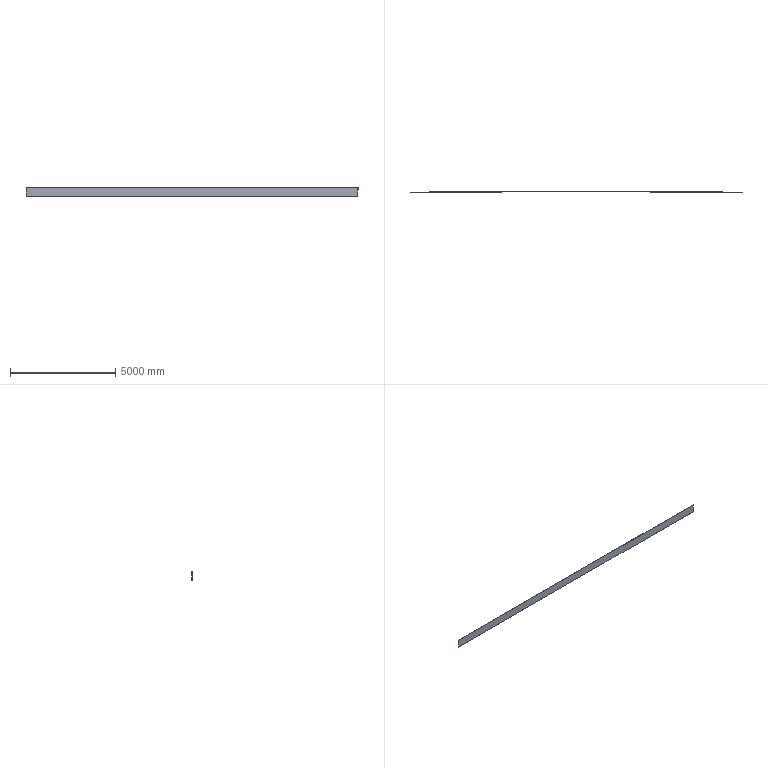Component | SolidWorks | LowerCover-1 | 1 solid | 6 faces | box 15785.09 x 28.11 x 400 mm | volume 63140405 mm3 | plane 4 | cylinder 2 | commonest cylinder face diameters 3440351.25 x1 3440371.25 x1 | material Plain Carbon Steel
STEP:
#1=CARTESIAN_POINT('',(34.151,97.311,80.917));
#2=VERTEX_POINT('',#1);
#3=CARTESIAN_POINT('',(34.151,97.311,65.169));
#4=VERTEX_POINT('',#3);
#5=CARTESIAN_POINT('',(34.151,97.311,65.169));
#6=DIRECTION('',(-0.,-0.,-1.));
#7=VECTOR('',#6,39.37);
#8=LINE('',#5,#7);
#9=EDGE_CURVE('',#2,#4,#8,.T.);
#10=ORIENTED_EDGE('',*,*,#9,.T.);
#11=CARTESIAN_POINT('',(655.608,97.311,65.169));
#12=VERTEX_POINT('',#11);
#13=CARTESIAN_POINT('',(344.879,-67625.426,65.169));
#14=DIRECTION('',(0.,0.,1.));
#15=DIRECTION('',(-1.,0.,0.));
#16=AXIS2_PLACEMENT_3D('',#13,#14,#15);
#17=CIRCLE('',#16,67723.45);
#18=EDGE_CURVE('',#12,#4,#17,.T.);
#19=ORIENTED_EDGE('',*,*,#18,.F.);
#20=CARTESIAN_POINT('',(655.608,97.311,80.917));
#21=VERTEX_POINT('',#20);
#22=CARTESIAN_POINT('',(655.608,97.311,65.169));
#23=DIRECTION('',(0.,0.,1.));
#24=VECTOR('',#23,39.37);
#25=LINE('',#22,#24);
#26=EDGE_CURVE('',#12,#21,#25,.T.);
#27=ORIENTED_EDGE('',*,*,#26,.T.);
#28=CARTESIAN_POINT('',(344.879,-67625.426,80.917));
#29=DIRECTION('',(0.,0.,1.));
#30=DIRECTION('',(-1.,0.,0.));
#31=AXIS2_PLACEMENT_3D('',#28,#29,#30);
#32=CIRCLE('',#31,67723.45);
#33=EDGE_CURVE('',#21,#2,#32,.T.);
#34=ORIENTED_EDGE('',*,*,#33,.T.);
#35=EDGE_LOOP('',(#10,#19,#27,#34));
#36=FACE_OUTER_BOUND('',#35,.T.);
#37=CARTESIAN_POINT('',(344.879,-67625.426,65.169));
#38=DIRECTION('',(0.,0.,1.));
#39=DIRECTION('',(1.,0.,-0.));
#40=AXIS2_PLACEMENT_3D('',#37,#38,#39);
#41=CYLINDRICAL_SURFACE('',#40,67723.45);
#42=ADVANCED_FACE('',(#36),#41,.F.);
#43=CARTESIAN_POINT('',(655.61,97.705,65.169));
#44=VERTEX_POINT('',#43);
#45=CARTESIAN_POINT('',(34.149,97.705,65.169));
#46=VERTEX_POINT('',#45);
#47=CARTESIAN_POINT('',(344.879,-67625.426,65.169));
#48=DIRECTION('',(0.,0.,1.));
#49=DIRECTION('',(1.,0.,-0.));
#50=AXIS2_PLACEMENT_3D('',#47,#48,#49);
#51=CIRCLE('',#50,67723.844);
#52=EDGE_CURVE('',#44,#46,#51,.T.);
#53=ORIENTED_EDGE('',*,*,#52,.T.);
#54=CARTESIAN_POINT('',(34.149,97.705,80.917));
#55=VERTEX_POINT('',#54);
#56=CARTESIAN_POINT('',(34.149,97.705,65.169));
#57=DIRECTION('',(-0.,-0.,-1.));
#58=VECTOR('',#57,39.37);
#59=LINE('',#56,#58);
#60=EDGE_CURVE('',#55,#46,#59,.T.);
#61=ORIENTED_EDGE('',*,*,#60,.F.);
#62=CARTESIAN_POINT('',(655.61,97.705,80.917));
#63=VERTEX_POINT('',#62);
#64=CARTESIAN_POINT('',(344.879,-67625.426,80.917));
#65=DIRECTION('',(0.,0.,1.));
#66=DIRECTION('',(1.,0.,-0.));
#67=AXIS2_PLACEMENT_3D('',#64,#65,#66);
#68=CIRCLE('',#67,67723.844);
#69=EDGE_CURVE('',#63,#55,#68,.T.);
#70=ORIENTED_EDGE('',*,*,#69,.F.);
#71=CARTESIAN_POINT('',(655.61,97.705,65.169));
#72=DIRECTION('',(0.,0.,1.));
#73=VECTOR('',#72,39.37);
#74=LINE('',#71,#73);
#75=EDGE_CURVE('',#44,#63,#74,.T.);
#76=ORIENTED_EDGE('',*,*,#75,.F.);
#77=EDGE_LOOP('',(#53,#61,#70,#76));
#78=FACE_OUTER_BOUND('',#77,.T.);
#79=CARTESIAN_POINT('',(344.879,-67625.426,65.169));
#80=DIRECTION('',(0.,0.,1.));
#81=DIRECTION('',(1.,0.,-0.));
#82=AXIS2_PLACEMENT_3D('',#79,#80,#81);
#83=CYLINDRICAL_SURFACE('',#82,67723.844);
#84=ADVANCED_FACE('',(#78),#83,.T.);
#85=ORIENTED_EDGE('',*,*,#18,.T.);
#86=CARTESIAN_POINT('',(34.151,97.311,65.169));
#87=DIRECTION('',(-0.004588,1.,0.));
#88=VECTOR('',#87,39.37);
#89=LINE('',#86,#88);
#90=EDGE_CURVE('',#4,#46,#89,.T.);
#91=ORIENTED_EDGE('',*,*,#90,.T.);
#92=ORIENTED_EDGE('',*,*,#52,.F.);
#93=CARTESIAN_POINT('',(655.608,97.311,65.169));
#94=DIRECTION('',(0.004588,1.,-0.));
#95=VECTOR('',#94,39.37);
#96=LINE('',#93,#95);
#97=EDGE_CURVE('',#12,#44,#96,.T.);
#98=ORIENTED_EDGE('',*,*,#97,.F.);
#99=EDGE_LOOP('',(#85,#91,#92,#98));
#100=FACE_OUTER_BOUND('',#99,.T.);
#101=CARTESIAN_POINT('',(344.879,-67625.426,65.169));
#102=DIRECTION('',(-0.,-0.,-1.));
#103=DIRECTION('',(-1.,-0.,0.));
#104=AXIS2_PLACEMENT_3D('',#101,#102,#103);
#105=PLANE('',#104);
#106=ADVANCED_FACE('',(#100),#105,.T.);
#107=CARTESIAN_POINT('',(34.151,97.311,80.917));
#108=DIRECTION('',(-0.004588,1.,0.));
#109=VECTOR('',#108,39.37);
#110=LINE('',#107,#109);
#111=EDGE_CURVE('',#2,#55,#110,.T.);
#112=ORIENTED_EDGE('',*,*,#111,.F.);
#113=ORIENTED_EDGE('',*,*,#33,.F.);
#114=CARTESIAN_POINT('',(655.608,97.311,80.917));
#115=DIRECTION('',(0.004588,1.,-0.));
#116=VECTOR('',#115,39.37);
#117=LINE('',#114,#116);
#118=EDGE_CURVE('',#21,#63,#117,.T.);
#119=ORIENTED_EDGE('',*,*,#118,.T.);
#120=ORIENTED_EDGE('',*,*,#69,.T.);
#121=EDGE_LOOP('',(#112,#113,#119,#120));
#122=FACE_OUTER_BOUND('',#121,.T.);
#123=CARTESIAN_POINT('',(344.879,-67625.426,80.917));
#124=DIRECTION('',(-0.,-0.,-1.));
#125=DIRECTION('',(-1.,-0.,0.));
#126=AXIS2_PLACEMENT_3D('',#123,#124,#125);
#127=PLANE('',#126);
#128=ADVANCED_FACE('',(#122),#127,.F.);
#129=ORIENTED_EDGE('',*,*,#118,.F.);
#130=ORIENTED_EDGE('',*,*,#26,.F.);
#131=ORIENTED_EDGE('',*,*,#97,.T.);
#132=ORIENTED_EDGE('',*,*,#75,.T.);
#133=EDGE_LOOP('',(#129,#130,#131,#132));
#134=FACE_OUTER_BOUND('',#133,.T.);
#135=CARTESIAN_POINT('',(655.608,97.311,73.043));
#136=DIRECTION('',(-1.,0.004588,0.));
#137=DIRECTION('',(0.,0.,1.));
#138=AXIS2_PLACEMENT_3D('',#135,#136,#137);
#139=PLANE('',#138);
#140=ADVANCED_FACE('',(#134),#139,.F.);
#141=ORIENTED_EDGE('',*,*,#90,.F.);
#142=ORIENTED_EDGE('',*,*,#9,.F.);
#143=ORIENTED_EDGE('',*,*,#111,.T.);
#144=ORIENTED_EDGE('',*,*,#60,.T.);
#145=EDGE_LOOP('',(#141,#142,#143,#144));
#146=FACE_OUTER_BOUND('',#145,.T.);
#147=CARTESIAN_POINT('',(34.151,97.311,73.043));
#148=DIRECTION('',(-1.,-0.004588,0.));
#149=DIRECTION('',(0.,0.,1.));
#150=AXIS2_PLACEMENT_3D('',#147,#148,#149);
#151=PLANE('',#150);
#152=ADVANCED_FACE('',(#146),#151,.T.);
#153=CLOSED_SHELL('',(#42,#84,#106,#128,#140,#152));
#154=MANIFOLD_SOLID_BREP('',#153);
#155=CARTESIAN_POINT('',(0.,0.,0.));
#156=DIRECTION('',(0.,0.,1.));
#157=DIRECTION('',(1.,0.,0.));
#158=AXIS2_PLACEMENT_3D('',#155,#156,#157);
#159=(LENGTH_UNIT()NAMED_UNIT(*)SI_UNIT($,.METRE.));
#160=LENGTH_MEASURE_WITH_UNIT(LENGTH_MEASURE(0.0254),#159);
#161=DIMENSIONAL_EXPONENTS(1.,0.,0.,0.,0.,0.,0.);
#162=(CONVERSION_BASED_UNIT('',#160)LENGTH_UNIT()NAMED_UNIT(#161));
#163=UNCERTAINTY_MEASURE_WITH_UNIT(LENGTH_MEASURE(0.00001),#162,'','');
#164=(NAMED_UNIT(*)PLANE_ANGLE_UNIT()SI_UNIT($,.RADIAN.));
#165=(NAMED_UNIT(*)SI_UNIT($,.STERADIAN.)SOLID_ANGLE_UNIT());
#166=(GEOMETRIC_REPRESENTATION_CONTEXT(3)GLOBAL_UNCERTAINTY_ASSIGNED_CONTEXT((#163))GLOBAL_UNIT_ASSIGNED_CONTEXT((#162,#164,#165))REPRESENTATION_CONTEXT('',''));
#167=ADVANCED_BREP_SHAPE_REPRESENTATION('',(#154,#158),#166);
#168=COLOUR_RGB('',0.7922,0.8196,0.9333);
#169=FILL_AREA_STYLE_COLOUR('',#168);
#170=FILL_AREA_STYLE('',(#169));
#171=SURFACE_STYLE_FILL_AREA(#170);
#172=SURFACE_SIDE_STYLE('',(#171));
#173=SURFACE_STYLE_USAGE(.BOTH.,#172);
#174=PRESENTATION_STYLE_ASSIGNMENT((#173));
#175=STYLED_ITEM('',(#174),#154);
#176=(LENGTH_UNIT()NAMED_UNIT(*)SI_UNIT($,.METRE.));
#177=LENGTH_MEASURE_WITH_UNIT(LENGTH_MEASURE(0.0254),#176);
#178=DIMENSIONAL_EXPONENTS(1.,0.,0.,0.,0.,0.,0.);
#179=(CONVERSION_BASED_UNIT('',#177)LENGTH_UNIT()NAMED_UNIT(#178));
#180=UNCERTAINTY_MEASURE_WITH_UNIT(LENGTH_MEASURE(0.00001),#179,'','');
#181=(NAMED_UNIT(*)PLANE_ANGLE_UNIT()SI_UNIT($,.RADIAN.));
#182=(NAMED_UNIT(*)SI_UNIT($,.STERADIAN.)SOLID_ANGLE_UNIT());
#183=(GEOMETRIC_REPRESENTATION_CONTEXT(3)GLOBAL_UNCERTAINTY_ASSIGNED_CONTEXT((#180))GLOBAL_UNIT_ASSIGNED_CONTEXT((#179,#181,#182))REPRESENTATION_CONTEXT('',''));
#184=MECHANICAL_DESIGN_GEOMETRIC_PRESENTATION_REPRESENTATION('',(#175),#183);
#185=PRESENTATION_LAYER_ASSIGNMENT('','',(#175));